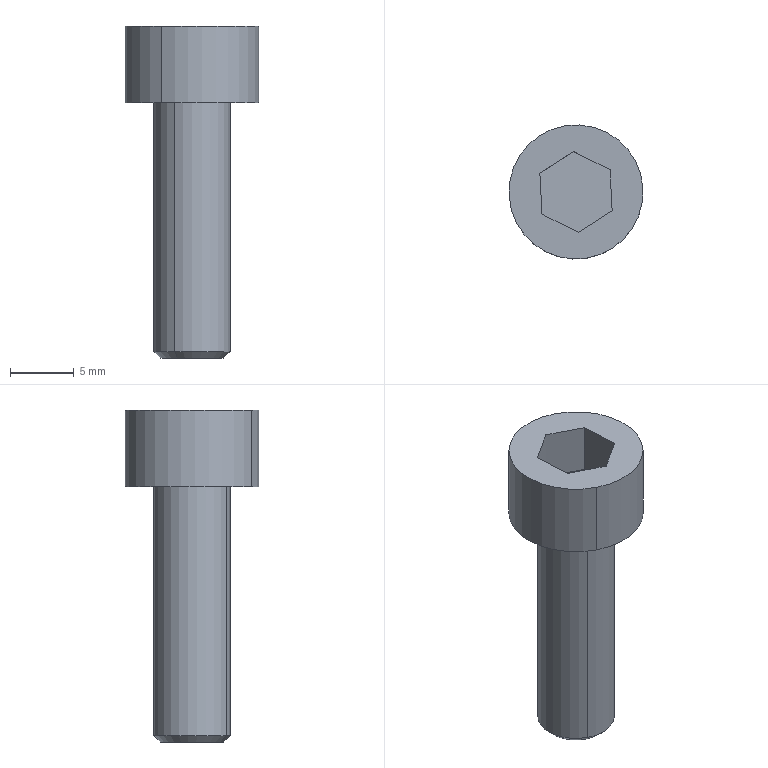Component | SolidWorks | M6x20HexSocketCap-2 | 1 solid | 16 faces | box 10.5 x 10.5 x 26 mm | volume 978 mm3 | plane 10 | cylinder 4 | cone 2 | commonest cylinder face diameters 6 x2 10.5 x2 | material #45
STEP:
#1=CARTESIAN_POINT('',(0.07331,12.286,-0.4488));
#2=VERTEX_POINT('',#1);
#3=CARTESIAN_POINT('',(0.1629,12.462,-0.4488));
#4=VERTEX_POINT('',#3);
#5=CARTESIAN_POINT('',(0.1181,12.374,-0.4488));
#6=DIRECTION('',(0.,0.,-1.));
#7=DIRECTION('',(-0.4552,-0.8904,0.));
#8=AXIS2_PLACEMENT_3D('',#5,#6,#7);
#9=CIRCLE('',#8,0.09843);
#10=EDGE_CURVE('',#2,#4,#9,.T.);
#11=ORIENTED_EDGE('',*,*,#10,.F.);
#12=CARTESIAN_POINT('',(0.06435,12.269,-0.4291));
#13=VERTEX_POINT('',#12);
#14=CARTESIAN_POINT('',(0.06435,12.269,-0.4291));
#15=DIRECTION('',(-0.3219,-0.6296,0.7071));
#16=VECTOR('',#15,39.37);
#17=LINE('',#14,#16);
#18=EDGE_CURVE('',#2,#13,#17,.T.);
#19=ORIENTED_EDGE('',*,*,#18,.T.);
#20=CARTESIAN_POINT('',(0.1719,12.479,-0.4291));
#21=VERTEX_POINT('',#20);
#22=CARTESIAN_POINT('',(0.1181,12.374,-0.4291));
#23=DIRECTION('',(0.,0.,-1.));
#24=DIRECTION('',(-0.4552,-0.8904,0.));
#25=AXIS2_PLACEMENT_3D('',#22,#23,#24);
#26=CIRCLE('',#25,0.1181);
#27=EDGE_CURVE('',#13,#21,#26,.T.);
#28=ORIENTED_EDGE('',*,*,#27,.T.);
#29=CARTESIAN_POINT('',(0.1719,12.479,-0.4291));
#30=DIRECTION('',(0.3219,0.6296,0.7071));
#31=VECTOR('',#30,39.37);
#32=LINE('',#29,#31);
#33=EDGE_CURVE('',#4,#21,#32,.T.);
#34=ORIENTED_EDGE('',*,*,#33,.F.);
#35=EDGE_LOOP('',(#11,#19,#28,#34));
#36=FACE_OUTER_BOUND('',#35,.T.);
#37=CARTESIAN_POINT('',(0.1181,12.374,-0.4291));
#38=DIRECTION('',(-0.,-0.,1.));
#39=DIRECTION('',(0.4552,0.8904,0.));
#40=AXIS2_PLACEMENT_3D('',#37,#38,#39);
#41=CONICAL_SURFACE('',#40,0.1181,0.7854);
#42=ADVANCED_FACE('',(#36),#41,.T.);
#43=CARTESIAN_POINT('',(0.06435,12.269,0.3386));
#44=VERTEX_POINT('',#43);
#45=CARTESIAN_POINT('',(0.1719,12.479,0.3386));
#46=VERTEX_POINT('',#45);
#47=CARTESIAN_POINT('',(0.1181,12.374,0.3386));
#48=DIRECTION('',(0.,0.,-1.));
#49=DIRECTION('',(-0.4552,-0.8904,0.));
#50=AXIS2_PLACEMENT_3D('',#47,#48,#49);
#51=CIRCLE('',#50,0.1181);
#52=EDGE_CURVE('',#44,#46,#51,.T.);
#53=ORIENTED_EDGE('',*,*,#52,.T.);
#54=CARTESIAN_POINT('',(0.1719,12.479,-0.4488));
#55=DIRECTION('',(0.,0.,-1.));
#56=VECTOR('',#55,39.37);
#57=LINE('',#54,#56);
#58=EDGE_CURVE('',#46,#21,#57,.T.);
#59=ORIENTED_EDGE('',*,*,#58,.T.);
#60=ORIENTED_EDGE('',*,*,#27,.F.);
#61=CARTESIAN_POINT('',(0.06435,12.269,-0.4488));
#62=DIRECTION('',(0.,0.,-1.));
#63=VECTOR('',#62,39.37);
#64=LINE('',#61,#63);
#65=EDGE_CURVE('',#44,#13,#64,.T.);
#66=ORIENTED_EDGE('',*,*,#65,.F.);
#67=EDGE_LOOP('',(#53,#59,#60,#66));
#68=FACE_OUTER_BOUND('',#67,.T.);
#69=CARTESIAN_POINT('',(0.1181,12.374,-0.4488));
#70=DIRECTION('',(0.,0.,-1.));
#71=DIRECTION('',(-0.4552,-0.8904,0.));
#72=AXIS2_PLACEMENT_3D('',#69,#70,#71);
#73=CYLINDRICAL_SURFACE('',#72,0.1181);
#74=ADVANCED_FACE('',(#68),#73,.T.);
#75=CARTESIAN_POINT('',(0.02403,12.19,0.5748));
#76=VERTEX_POINT('',#75);
#77=CARTESIAN_POINT('',(0.2122,12.558,0.5748));
#78=VERTEX_POINT('',#77);
#79=CARTESIAN_POINT('',(0.1181,12.374,0.5748));
#80=DIRECTION('',(0.,0.,-1.));
#81=DIRECTION('',(-0.4552,-0.8904,0.));
#82=AXIS2_PLACEMENT_3D('',#79,#80,#81);
#83=CIRCLE('',#82,0.2067);
#84=EDGE_CURVE('',#76,#78,#83,.T.);
#85=ORIENTED_EDGE('',*,*,#84,.T.);
#86=CARTESIAN_POINT('',(0.2122,12.558,0.3386));
#87=VERTEX_POINT('',#86);
#88=CARTESIAN_POINT('',(0.2122,12.558,-0.4488));
#89=DIRECTION('',(0.,0.,-1.));
#90=VECTOR('',#89,39.37);
#91=LINE('',#88,#90);
#92=EDGE_CURVE('',#78,#87,#91,.T.);
#93=ORIENTED_EDGE('',*,*,#92,.T.);
#94=CARTESIAN_POINT('',(0.02403,12.19,0.3386));
#95=VERTEX_POINT('',#94);
#96=CARTESIAN_POINT('',(0.1181,12.374,0.3386));
#97=DIRECTION('',(0.,0.,-1.));
#98=DIRECTION('',(-0.4552,-0.8904,0.));
#99=AXIS2_PLACEMENT_3D('',#96,#97,#98);
#100=CIRCLE('',#99,0.2067);
#101=EDGE_CURVE('',#95,#87,#100,.T.);
#102=ORIENTED_EDGE('',*,*,#101,.F.);
#103=CARTESIAN_POINT('',(0.02403,12.19,-0.4488));
#104=DIRECTION('',(0.,0.,-1.));
#105=VECTOR('',#104,39.37);
#106=LINE('',#103,#105);
#107=EDGE_CURVE('',#76,#95,#106,.T.);
#108=ORIENTED_EDGE('',*,*,#107,.F.);
#109=EDGE_LOOP('',(#85,#93,#102,#108));
#110=FACE_OUTER_BOUND('',#109,.T.);
#111=CARTESIAN_POINT('',(0.1181,12.374,-0.4488));
#112=DIRECTION('',(0.,0.,-1.));
#113=DIRECTION('',(-0.4552,-0.8904,0.));
#114=AXIS2_PLACEMENT_3D('',#111,#112,#113);
#115=CYLINDRICAL_SURFACE('',#114,0.2067);
#116=ADVANCED_FACE('',(#110),#115,.T.);
#117=CARTESIAN_POINT('',(0.006795,12.431,0.5748));
#118=VERTEX_POINT('',#117);
#119=CARTESIAN_POINT('',(0.01317,12.306,0.5748));
#120=VERTEX_POINT('',#119);
#121=CARTESIAN_POINT('',(0.006795,12.431,0.5748));
#122=DIRECTION('',(0.05102,-0.9987,-0.));
#123=VECTOR('',#122,39.37);
#124=LINE('',#121,#123);
#125=EDGE_CURVE('',#118,#120,#124,.T.);
#126=ORIENTED_EDGE('',*,*,#125,.F.);
#127=CARTESIAN_POINT('',(0.1117,12.499,0.5748));
#128=VERTEX_POINT('',#127);
#129=CARTESIAN_POINT('',(0.1117,12.499,0.5748));
#130=DIRECTION('',(-0.8394,-0.5435,-0.));
#131=VECTOR('',#130,39.37);
#132=LINE('',#129,#131);
#133=EDGE_CURVE('',#128,#118,#132,.T.);
#134=ORIENTED_EDGE('',*,*,#133,.F.);
#135=CARTESIAN_POINT('',(0.223,12.442,0.5748));
#136=VERTEX_POINT('',#135);
#137=CARTESIAN_POINT('',(0.223,12.442,0.5748));
#138=DIRECTION('',(-0.8904,0.4552,0.));
#139=VECTOR('',#138,39.37);
#140=LINE('',#137,#139);
#141=EDGE_CURVE('',#136,#128,#140,.T.);
#142=ORIENTED_EDGE('',*,*,#141,.F.);
#143=CARTESIAN_POINT('',(0.2294,12.317,0.5748));
#144=VERTEX_POINT('',#143);
#145=CARTESIAN_POINT('',(0.2294,12.317,0.5748));
#146=DIRECTION('',(-0.05102,0.9987,0.));
#147=VECTOR('',#146,39.37);
#148=LINE('',#145,#147);
#149=EDGE_CURVE('',#144,#136,#148,.T.);
#150=ORIENTED_EDGE('',*,*,#149,.F.);
#151=CARTESIAN_POINT('',(0.1245,12.249,0.5748));
#152=VERTEX_POINT('',#151);
#153=CARTESIAN_POINT('',(0.1245,12.249,0.5748));
#154=DIRECTION('',(0.8394,0.5435,0.));
#155=VECTOR('',#154,39.37);
#156=LINE('',#153,#155);
#157=EDGE_CURVE('',#152,#144,#156,.T.);
#158=ORIENTED_EDGE('',*,*,#157,.F.);
#159=CARTESIAN_POINT('',(0.01317,12.306,0.5748));
#160=DIRECTION('',(0.8904,-0.4552,-0.));
#161=VECTOR('',#160,39.37);
#162=LINE('',#159,#161);
#163=EDGE_CURVE('',#120,#152,#162,.T.);
#164=ORIENTED_EDGE('',*,*,#163,.F.);
#165=EDGE_LOOP('',(#126,#134,#142,#150,#158,#164));
#166=FACE_BOUND('',#165,.T.);
#167=ORIENTED_EDGE('',*,*,#84,.F.);
#168=CARTESIAN_POINT('',(0.1181,12.374,0.5748));
#169=DIRECTION('',(0.,0.,-1.));
#170=DIRECTION('',(-0.4552,-0.8904,0.));
#171=AXIS2_PLACEMENT_3D('',#168,#169,#170);
#172=CIRCLE('',#171,0.2067);
#173=EDGE_CURVE('',#78,#76,#172,.T.);
#174=ORIENTED_EDGE('',*,*,#173,.F.);
#175=EDGE_LOOP('',(#167,#174));
#176=FACE_OUTER_BOUND('',#175,.T.);
#177=CARTESIAN_POINT('',(0.1181,12.374,0.5748));
#178=DIRECTION('',(0.,0.,-1.));
#179=DIRECTION('',(-0.4552,-0.8904,-0.));
#180=AXIS2_PLACEMENT_3D('',#177,#178,#179);
#181=PLANE('',#180);
#182=ADVANCED_FACE('',(#166,#176),#181,.F.);
#183=ORIENTED_EDGE('',*,*,#92,.F.);
#184=ORIENTED_EDGE('',*,*,#173,.T.);
#185=ORIENTED_EDGE('',*,*,#107,.T.);
#186=CARTESIAN_POINT('',(0.1181,12.374,0.3386));
#187=DIRECTION('',(0.,0.,-1.));
#188=DIRECTION('',(-0.4552,-0.8904,0.));
#189=AXIS2_PLACEMENT_3D('',#186,#187,#188);
#190=CIRCLE('',#189,0.2067);
#191=EDGE_CURVE('',#87,#95,#190,.T.);
#192=ORIENTED_EDGE('',*,*,#191,.F.);
#193=EDGE_LOOP('',(#183,#184,#185,#192));
#194=FACE_OUTER_BOUND('',#193,.T.);
#195=CARTESIAN_POINT('',(0.1181,12.374,-0.4488));
#196=DIRECTION('',(0.,0.,-1.));
#197=DIRECTION('',(-0.4552,-0.8904,0.));
#198=AXIS2_PLACEMENT_3D('',#195,#196,#197);
#199=CYLINDRICAL_SURFACE('',#198,0.2067);
#200=ADVANCED_FACE('',(#194),#199,.T.);
#201=ORIENTED_EDGE('',*,*,#52,.F.);
#202=CARTESIAN_POINT('',(0.1181,12.374,0.3386));
#203=DIRECTION('',(0.,0.,-1.));
#204=DIRECTION('',(-0.4552,-0.8904,0.));
#205=AXIS2_PLACEMENT_3D('',#202,#203,#204);
#206=CIRCLE('',#205,0.1181);
#207=EDGE_CURVE('',#46,#44,#206,.T.);
#208=ORIENTED_EDGE('',*,*,#207,.F.);
#209=EDGE_LOOP('',(#201,#208));
#210=FACE_BOUND('',#209,.T.);
#211=ORIENTED_EDGE('',*,*,#101,.T.);
#212=ORIENTED_EDGE('',*,*,#191,.T.);
#213=EDGE_LOOP('',(#211,#212));
#214=FACE_OUTER_BOUND('',#213,.T.);
#215=CARTESIAN_POINT('',(0.2122,12.558,0.3386));
#216=DIRECTION('',(-0.,-0.,1.));
#217=DIRECTION('',(0.4552,0.8904,0.));
#218=AXIS2_PLACEMENT_3D('',#215,#216,#217);
#219=PLANE('',#218);
#220=ADVANCED_FACE('',(#210,#214),#219,.F.);
#221=ORIENTED_EDGE('',*,*,#58,.F.);
#222=ORIENTED_EDGE('',*,*,#207,.T.);
#223=ORIENTED_EDGE('',*,*,#65,.T.);
#224=CARTESIAN_POINT('',(0.1181,12.374,-0.4291));
#225=DIRECTION('',(0.,0.,-1.));
#226=DIRECTION('',(-0.4552,-0.8904,0.));
#227=AXIS2_PLACEMENT_3D('',#224,#225,#226);
#228=CIRCLE('',#227,0.1181);
#229=EDGE_CURVE('',#21,#13,#228,.T.);
#230=ORIENTED_EDGE('',*,*,#229,.F.);
#231=EDGE_LOOP('',(#221,#222,#223,#230));
#232=FACE_OUTER_BOUND('',#231,.T.);
#233=CARTESIAN_POINT('',(0.1181,12.374,-0.4488));
#234=DIRECTION('',(0.,0.,-1.));
#235=DIRECTION('',(-0.4552,-0.8904,0.));
#236=AXIS2_PLACEMENT_3D('',#233,#234,#235);
#237=CYLINDRICAL_SURFACE('',#236,0.1181);
#238=ADVANCED_FACE('',(#232),#237,.T.);
#239=ORIENTED_EDGE('',*,*,#18,.F.);
#240=CARTESIAN_POINT('',(0.1181,12.374,-0.4488));
#241=DIRECTION('',(0.,0.,-1.));
#242=DIRECTION('',(-0.4552,-0.8904,0.));
#243=AXIS2_PLACEMENT_3D('',#240,#241,#242);
#244=CIRCLE('',#243,0.09843);
#245=EDGE_CURVE('',#4,#2,#244,.T.);
#246=ORIENTED_EDGE('',*,*,#245,.F.);
#247=ORIENTED_EDGE('',*,*,#33,.T.);
#248=ORIENTED_EDGE('',*,*,#229,.T.);
#249=EDGE_LOOP('',(#239,#246,#247,#248));
#250=FACE_OUTER_BOUND('',#249,.T.);
#251=CARTESIAN_POINT('',(0.1181,12.374,-0.4291));
#252=DIRECTION('',(-0.,-0.,1.));
#253=DIRECTION('',(0.4552,0.8904,0.));
#254=AXIS2_PLACEMENT_3D('',#251,#252,#253);
#255=CONICAL_SURFACE('',#254,0.1181,0.7854);
#256=ADVANCED_FACE('',(#250),#255,.T.);
#257=ORIENTED_EDGE('',*,*,#245,.T.);
#258=ORIENTED_EDGE('',*,*,#10,.T.);
#259=EDGE_LOOP('',(#257,#258));
#260=FACE_OUTER_BOUND('',#259,.T.);
#261=CARTESIAN_POINT('',(0.1629,12.462,-0.4488));
#262=DIRECTION('',(-0.,-0.,1.));
#263=DIRECTION('',(0.4552,0.8904,0.));
#264=AXIS2_PLACEMENT_3D('',#261,#262,#263);
#265=PLANE('',#264);
#266=ADVANCED_FACE('',(#260),#265,.F.);
#267=ORIENTED_EDGE('',*,*,#133,.T.);
#268=CARTESIAN_POINT('',(0.006795,12.431,0.4173));
#269=VERTEX_POINT('',#268);
#270=CARTESIAN_POINT('',(0.006795,12.431,0.4173));
#271=DIRECTION('',(-0.,-0.,1.));
#272=VECTOR('',#271,39.37);
#273=LINE('',#270,#272);
#274=EDGE_CURVE('',#269,#118,#273,.T.);
#275=ORIENTED_EDGE('',*,*,#274,.F.);
#276=CARTESIAN_POINT('',(0.1117,12.499,0.4173));
#277=VERTEX_POINT('',#276);
#278=CARTESIAN_POINT('',(0.1117,12.499,0.4173));
#279=DIRECTION('',(-0.8394,-0.5435,-0.));
#280=VECTOR('',#279,39.37);
#281=LINE('',#278,#280);
#282=EDGE_CURVE('',#277,#269,#281,.T.);
#283=ORIENTED_EDGE('',*,*,#282,.F.);
#284=CARTESIAN_POINT('',(0.1117,12.499,0.4173));
#285=DIRECTION('',(-0.,-0.,1.));
#286=VECTOR('',#285,39.37);
#287=LINE('',#284,#286);
#288=EDGE_CURVE('',#277,#128,#287,.T.);
#289=ORIENTED_EDGE('',*,*,#288,.T.);
#290=EDGE_LOOP('',(#267,#275,#283,#289));
#291=FACE_OUTER_BOUND('',#290,.T.);
#292=CARTESIAN_POINT('',(0.1117,12.499,0.4173));
#293=DIRECTION('',(-0.5435,0.8394,0.));
#294=DIRECTION('',(0.8394,0.5435,0.));
#295=AXIS2_PLACEMENT_3D('',#292,#293,#294);
#296=PLANE('',#295);
#297=ADVANCED_FACE('',(#291),#296,.F.);
#298=ORIENTED_EDGE('',*,*,#141,.T.);
#299=ORIENTED_EDGE('',*,*,#288,.F.);
#300=CARTESIAN_POINT('',(0.223,12.442,0.4173));
#301=VERTEX_POINT('',#300);
#302=CARTESIAN_POINT('',(0.223,12.442,0.4173));
#303=DIRECTION('',(-0.8904,0.4552,0.));
#304=VECTOR('',#303,39.37);
#305=LINE('',#302,#304);
#306=EDGE_CURVE('',#301,#277,#305,.T.);
#307=ORIENTED_EDGE('',*,*,#306,.F.);
#308=CARTESIAN_POINT('',(0.223,12.442,0.4173));
#309=DIRECTION('',(-0.,-0.,1.));
#310=VECTOR('',#309,39.37);
#311=LINE('',#308,#310);
#312=EDGE_CURVE('',#301,#136,#311,.T.);
#313=ORIENTED_EDGE('',*,*,#312,.T.);
#314=EDGE_LOOP('',(#298,#299,#307,#313));
#315=FACE_OUTER_BOUND('',#314,.T.);
#316=CARTESIAN_POINT('',(0.223,12.442,0.4173));
#317=DIRECTION('',(0.4552,0.8904,0.));
#318=DIRECTION('',(0.,0.,-1.));
#319=AXIS2_PLACEMENT_3D('',#316,#317,#318);
#320=PLANE('',#319);
#321=ADVANCED_FACE('',(#315),#320,.F.);
#322=ORIENTED_EDGE('',*,*,#149,.T.);
#323=ORIENTED_EDGE('',*,*,#312,.F.);
#324=CARTESIAN_POINT('',(0.2294,12.317,0.4173));
#325=VERTEX_POINT('',#324);
#326=CARTESIAN_POINT('',(0.2294,12.317,0.4173));
#327=DIRECTION('',(-0.05102,0.9987,0.));
#328=VECTOR('',#327,39.37);
#329=LINE('',#326,#328);
#330=EDGE_CURVE('',#325,#301,#329,.T.);
#331=ORIENTED_EDGE('',*,*,#330,.F.);
#332=CARTESIAN_POINT('',(0.2294,12.317,0.4173));
#333=DIRECTION('',(-0.,-0.,1.));
#334=VECTOR('',#333,39.37);
#335=LINE('',#332,#334);
#336=EDGE_CURVE('',#325,#144,#335,.T.);
#337=ORIENTED_EDGE('',*,*,#336,.T.);
#338=EDGE_LOOP('',(#322,#323,#331,#337));
#339=FACE_OUTER_BOUND('',#338,.T.);
#340=CARTESIAN_POINT('',(0.2294,12.317,0.4173));
#341=DIRECTION('',(0.9987,0.05102,0.));
#342=DIRECTION('',(0.05102,-0.9987,-0.));
#343=AXIS2_PLACEMENT_3D('',#340,#341,#342);
#344=PLANE('',#343);
#345=ADVANCED_FACE('',(#339),#344,.F.);
#346=ORIENTED_EDGE('',*,*,#157,.T.);
#347=ORIENTED_EDGE('',*,*,#336,.F.);
#348=CARTESIAN_POINT('',(0.1245,12.249,0.4173));
#349=VERTEX_POINT('',#348);
#350=CARTESIAN_POINT('',(0.1245,12.249,0.4173));
#351=DIRECTION('',(0.8394,0.5435,0.));
#352=VECTOR('',#351,39.37);
#353=LINE('',#350,#352);
#354=EDGE_CURVE('',#349,#325,#353,.T.);
#355=ORIENTED_EDGE('',*,*,#354,.F.);
#356=CARTESIAN_POINT('',(0.1245,12.249,0.4173));
#357=DIRECTION('',(-0.,-0.,1.));
#358=VECTOR('',#357,39.37);
#359=LINE('',#356,#358);
#360=EDGE_CURVE('',#349,#152,#359,.T.);
#361=ORIENTED_EDGE('',*,*,#360,.T.);
#362=EDGE_LOOP('',(#346,#347,#355,#361));
#363=FACE_OUTER_BOUND('',#362,.T.);
#364=CARTESIAN_POINT('',(0.1245,12.249,0.4173));
#365=DIRECTION('',(0.5435,-0.8394,-0.));
#366=DIRECTION('',(-0.8394,-0.5435,-0.));
#367=AXIS2_PLACEMENT_3D('',#364,#365,#366);
#368=PLANE('',#367);
#369=ADVANCED_FACE('',(#363),#368,.F.);
#370=ORIENTED_EDGE('',*,*,#163,.T.);
#371=ORIENTED_EDGE('',*,*,#360,.F.);
#372=CARTESIAN_POINT('',(0.01317,12.306,0.4173));
#373=VERTEX_POINT('',#372);
#374=CARTESIAN_POINT('',(0.01317,12.306,0.4173));
#375=DIRECTION('',(0.8904,-0.4552,-0.));
#376=VECTOR('',#375,39.37);
#377=LINE('',#374,#376);
#378=EDGE_CURVE('',#373,#349,#377,.T.);
#379=ORIENTED_EDGE('',*,*,#378,.F.);
#380=CARTESIAN_POINT('',(0.01317,12.306,0.4173));
#381=DIRECTION('',(-0.,-0.,1.));
#382=VECTOR('',#381,39.37);
#383=LINE('',#380,#382);
#384=EDGE_CURVE('',#373,#120,#383,.T.);
#385=ORIENTED_EDGE('',*,*,#384,.T.);
#386=EDGE_LOOP('',(#370,#371,#379,#385));
#387=FACE_OUTER_BOUND('',#386,.T.);
#388=CARTESIAN_POINT('',(0.01317,12.306,0.4173));
#389=DIRECTION('',(-0.4552,-0.8904,-0.));
#390=DIRECTION('',(-0.,-0.,1.));
#391=AXIS2_PLACEMENT_3D('',#388,#389,#390);
#392=PLANE('',#391);
#393=ADVANCED_FACE('',(#387),#392,.F.);
#394=ORIENTED_EDGE('',*,*,#125,.T.);
#395=ORIENTED_EDGE('',*,*,#384,.F.);
#396=CARTESIAN_POINT('',(0.006795,12.431,0.4173));
#397=DIRECTION('',(0.05102,-0.9987,-0.));
#398=VECTOR('',#397,39.37);
#399=LINE('',#396,#398);
#400=EDGE_CURVE('',#269,#373,#399,.T.);
#401=ORIENTED_EDGE('',*,*,#400,.F.);
#402=ORIENTED_EDGE('',*,*,#274,.T.);
#403=EDGE_LOOP('',(#394,#395,#401,#402));
#404=FACE_OUTER_BOUND('',#403,.T.);
#405=CARTESIAN_POINT('',(0.006795,12.431,0.4173));
#406=DIRECTION('',(-0.9987,-0.05102,-0.));
#407=DIRECTION('',(-0.05102,0.9987,0.));
#408=AXIS2_PLACEMENT_3D('',#405,#406,#407);
#409=PLANE('',#408);
#410=ADVANCED_FACE('',(#404),#409,.F.);
#411=ORIENTED_EDGE('',*,*,#282,.T.);
#412=ORIENTED_EDGE('',*,*,#400,.T.);
#413=ORIENTED_EDGE('',*,*,#378,.T.);
#414=ORIENTED_EDGE('',*,*,#354,.T.);
#415=ORIENTED_EDGE('',*,*,#330,.T.);
#416=ORIENTED_EDGE('',*,*,#306,.T.);
#417=EDGE_LOOP('',(#411,#412,#413,#414,#415,#416));
#418=FACE_OUTER_BOUND('',#417,.T.);
#419=CARTESIAN_POINT('',(0.1181,12.374,0.4173));
#420=DIRECTION('',(-0.,-0.,1.));
#421=DIRECTION('',(0.4552,0.8904,0.));
#422=AXIS2_PLACEMENT_3D('',#419,#420,#421);
#423=PLANE('',#422);
#424=ADVANCED_FACE('',(#418),#423,.T.);
#425=CLOSED_SHELL('',(#42,#74,#116,#182,#200,#220,#238,#256,#266,#297,#321,#345,#369,#393,#410,#424));
#426=MANIFOLD_SOLID_BREP('',#425);
#427=CARTESIAN_POINT('',(0.,0.,0.));
#428=DIRECTION('',(0.,0.,1.));
#429=DIRECTION('',(1.,0.,0.));
#430=AXIS2_PLACEMENT_3D('',#427,#428,#429);
#431=(LENGTH_UNIT()NAMED_UNIT(*)SI_UNIT($,.METRE.));
#432=LENGTH_MEASURE_WITH_UNIT(LENGTH_MEASURE(0.0254),#431);
#433=DIMENSIONAL_EXPONENTS(1.,0.,0.,0.,0.,0.,0.);
#434=(CONVERSION_BASED_UNIT('',#432)LENGTH_UNIT()NAMED_UNIT(#433));
#435=UNCERTAINTY_MEASURE_WITH_UNIT(LENGTH_MEASURE(0.00001),#434,'','');
#436=(NAMED_UNIT(*)PLANE_ANGLE_UNIT()SI_UNIT($,.RADIAN.));
#437=(NAMED_UNIT(*)SI_UNIT($,.STERADIAN.)SOLID_ANGLE_UNIT());
#438=(GEOMETRIC_REPRESENTATION_CONTEXT(3)GLOBAL_UNCERTAINTY_ASSIGNED_CONTEXT((#435))GLOBAL_UNIT_ASSIGNED_CONTEXT((#434,#436,#437))REPRESENTATION_CONTEXT('',''));
#439=ADVANCED_BREP_SHAPE_REPRESENTATION('',(#426,#430),#438);
#440=COLOUR_RGB('',0.7922,0.8196,0.9333);
#441=FILL_AREA_STYLE_COLOUR('',#440);
#442=FILL_AREA_STYLE('',(#441));
#443=SURFACE_STYLE_FILL_AREA(#442);
#444=SURFACE_SIDE_STYLE('',(#443));
#445=SURFACE_STYLE_USAGE(.BOTH.,#444);
#446=PRESENTATION_STYLE_ASSIGNMENT((#445));
#447=STYLED_ITEM('',(#446),#426);
#448=PRESENTATION_LAYER_ASSIGNMENT('','',(#447));
#449=(LENGTH_UNIT()NAMED_UNIT(*)SI_UNIT($,.METRE.));
#450=LENGTH_MEASURE_WITH_UNIT(LENGTH_MEASURE(0.0254),#449);
#451=DIMENSIONAL_EXPONENTS(1.,0.,0.,0.,0.,0.,0.);
#452=(CONVERSION_BASED_UNIT('',#450)LENGTH_UNIT()NAMED_UNIT(#451));
#453=UNCERTAINTY_MEASURE_WITH_UNIT(LENGTH_MEASURE(0.00001),#452,'','');
#454=(NAMED_UNIT(*)PLANE_ANGLE_UNIT()SI_UNIT($,.RADIAN.));
#455=(NAMED_UNIT(*)SI_UNIT($,.STERADIAN.)SOLID_ANGLE_UNIT());
#456=(GEOMETRIC_REPRESENTATION_CONTEXT(3)GLOBAL_UNCERTAINTY_ASSIGNED_CONTEXT((#453))GLOBAL_UNIT_ASSIGNED_CONTEXT((#452,#454,#455))REPRESENTATION_CONTEXT('',''));
#457=MECHANICAL_DESIGN_GEOMETRIC_PRESENTATION_REPRESENTATION('',(#447),#456);